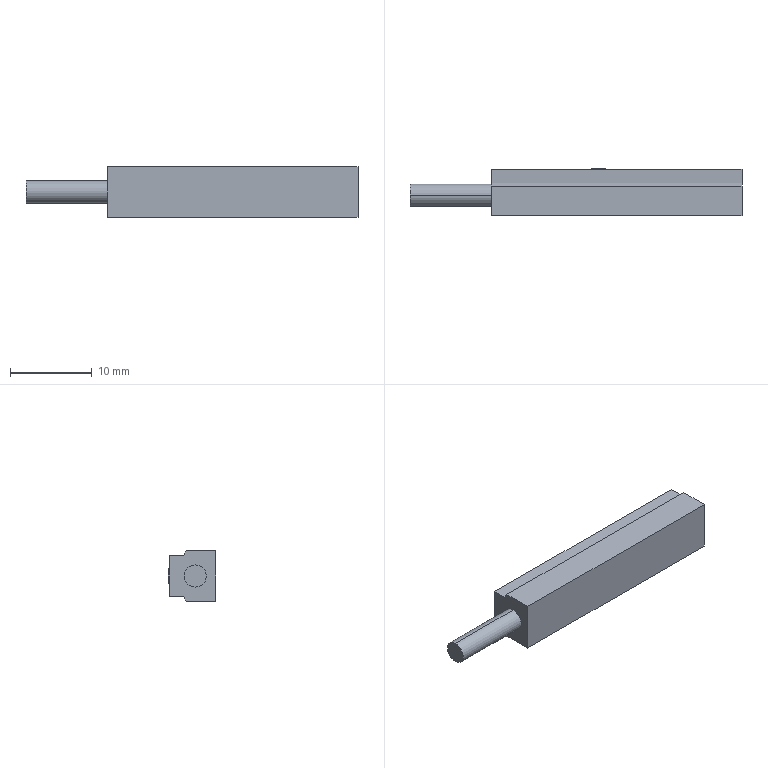Component | SolidWorks | F-YBExport-1-1_F-YBXCXSM10-15-Z73L-1_F-YBXCXSM10-15-Z73L_CXSSwitches(Z73)-1 | 1 solid | 33 faces | box 40.5 x 5.8 x 6.2 mm | volume 1063 mm3 | plane 27 | cylinder 6 | commonest cylinder face diameters 2.347 x2 2.5 x2 2.7 x2
STEP:
#1=COLOUR_RGB('',0.7922,0.8196,0.9333);
#2=FILL_AREA_STYLE_COLOUR('',#1);
#3=FILL_AREA_STYLE('',(#2));
#4=SURFACE_STYLE_FILL_AREA(#3);
#5=SURFACE_SIDE_STYLE('',(#4));
#6=SURFACE_STYLE_USAGE(.BOTH.,#5);
#7=PRESENTATION_STYLE_ASSIGNMENT((#6));
#8=CARTESIAN_POINT('',(13.609,14.688,6.265));
#9=VERTEX_POINT('',#8);
#10=CARTESIAN_POINT('',(13.537,14.688,6.227));
#11=VERTEX_POINT('',#10);
#12=CARTESIAN_POINT('',(13.563,14.688,6.265));
#13=DIRECTION('',(-0.,1.,0.));
#14=DIRECTION('',(1.,0.,0.));
#15=AXIS2_PLACEMENT_3D('',#12,#13,#14);
#16=CIRCLE('',#15,0.04621);
#17=EDGE_CURVE('',#9,#11,#16,.T.);
#18=ORIENTED_EDGE('',*,*,#17,.F.);
#19=CARTESIAN_POINT('',(13.609,14.648,6.265));
#20=VERTEX_POINT('',#19);
#21=CARTESIAN_POINT('',(13.609,14.688,6.265));
#22=DIRECTION('',(0.,-1.,-0.));
#23=VECTOR('',#22,39.37);
#24=LINE('',#21,#23);
#25=EDGE_CURVE('',#9,#20,#24,.T.);
#26=ORIENTED_EDGE('',*,*,#25,.T.);
#27=CARTESIAN_POINT('',(13.517,14.648,6.265));
#28=VERTEX_POINT('',#27);
#29=CARTESIAN_POINT('',(13.563,14.648,6.265));
#30=DIRECTION('',(-0.,1.,0.));
#31=DIRECTION('',(1.,0.,0.));
#32=AXIS2_PLACEMENT_3D('',#29,#30,#31);
#33=CIRCLE('',#32,0.04621);
#34=EDGE_CURVE('',#20,#28,#33,.T.);
#35=ORIENTED_EDGE('',*,*,#34,.T.);
#36=CARTESIAN_POINT('',(13.517,14.688,6.265));
#37=VERTEX_POINT('',#36);
#38=CARTESIAN_POINT('',(13.517,14.688,6.265));
#39=DIRECTION('',(0.,-1.,-0.));
#40=VECTOR('',#39,39.37);
#41=LINE('',#38,#40);
#42=EDGE_CURVE('',#37,#28,#41,.T.);
#43=ORIENTED_EDGE('',*,*,#42,.F.);
#44=CARTESIAN_POINT('',(13.525,14.688,6.239));
#45=VERTEX_POINT('',#44);
#46=CARTESIAN_POINT('',(13.563,14.688,6.265));
#47=DIRECTION('',(-0.,1.,0.));
#48=DIRECTION('',(1.,0.,0.));
#49=AXIS2_PLACEMENT_3D('',#46,#47,#48);
#50=CIRCLE('',#49,0.04621);
#51=EDGE_CURVE('',#45,#37,#50,.T.);
#52=ORIENTED_EDGE('',*,*,#51,.F.);
#53=CARTESIAN_POINT('',(13.525,14.668,6.239));
#54=VERTEX_POINT('',#53);
#55=CARTESIAN_POINT('',(13.525,14.688,6.239));
#56=DIRECTION('',(0.,-1.,-0.));
#57=VECTOR('',#56,39.37);
#58=LINE('',#55,#57);
#59=EDGE_CURVE('',#45,#54,#58,.T.);
#60=ORIENTED_EDGE('',*,*,#59,.T.);
#61=CARTESIAN_POINT('',(13.537,14.668,6.227));
#62=VERTEX_POINT('',#61);
#63=CARTESIAN_POINT('',(13.563,14.668,6.265));
#64=DIRECTION('',(-0.,1.,0.));
#65=DIRECTION('',(1.,0.,0.));
#66=AXIS2_PLACEMENT_3D('',#63,#64,#65);
#67=CIRCLE('',#66,0.04621);
#68=EDGE_CURVE('',#62,#54,#67,.T.);
#69=ORIENTED_EDGE('',*,*,#68,.F.);
#70=CARTESIAN_POINT('',(13.537,14.688,6.227));
#71=DIRECTION('',(-0.,1.,0.));
#72=VECTOR('',#71,39.37);
#73=LINE('',#70,#72);
#74=EDGE_CURVE('',#62,#11,#73,.T.);
#75=ORIENTED_EDGE('',*,*,#74,.T.);
#76=EDGE_LOOP('',(#18,#26,#35,#43,#52,#60,#69,#75));
#77=FACE_OUTER_BOUND('',#76,.T.);
#78=CARTESIAN_POINT('',(13.563,14.688,6.265));
#79=DIRECTION('',(0.,-1.,-0.));
#80=DIRECTION('',(-1.,0.,0.));
#81=AXIS2_PLACEMENT_3D('',#78,#79,#80);
#82=CYLINDRICAL_SURFACE('',#81,0.04621);
#83=ADVANCED_FACE('',(#77),#82,.T.);
#84=CARTESIAN_POINT('',(13.514,14.648,6.265));
#85=VERTEX_POINT('',#84);
#86=CARTESIAN_POINT('',(13.612,14.648,6.265));
#87=VERTEX_POINT('',#86);
#88=CARTESIAN_POINT('',(13.563,14.648,6.265));
#89=DIRECTION('',(-0.,1.,0.));
#90=DIRECTION('',(1.,0.,0.));
#91=AXIS2_PLACEMENT_3D('',#88,#89,#90);
#92=CIRCLE('',#91,0.04921);
#93=EDGE_CURVE('',#85,#87,#92,.T.);
#94=ORIENTED_EDGE('',*,*,#93,.F.);
#95=CARTESIAN_POINT('',(13.514,14.688,6.265));
#96=VERTEX_POINT('',#95);
#97=CARTESIAN_POINT('',(13.514,14.648,6.265));
#98=DIRECTION('',(-0.,1.,0.));
#99=VECTOR('',#98,39.37);
#100=LINE('',#97,#99);
#101=EDGE_CURVE('',#85,#96,#100,.T.);
#102=ORIENTED_EDGE('',*,*,#101,.T.);
#103=CARTESIAN_POINT('',(13.612,14.688,6.265));
#104=VERTEX_POINT('',#103);
#105=CARTESIAN_POINT('',(13.563,14.688,6.265));
#106=DIRECTION('',(-0.,1.,0.));
#107=DIRECTION('',(1.,0.,0.));
#108=AXIS2_PLACEMENT_3D('',#105,#106,#107);
#109=CIRCLE('',#108,0.04921);
#110=EDGE_CURVE('',#96,#104,#109,.T.);
#111=ORIENTED_EDGE('',*,*,#110,.T.);
#112=CARTESIAN_POINT('',(13.612,14.648,6.265));
#113=DIRECTION('',(-0.,1.,0.));
#114=VECTOR('',#113,39.37);
#115=LINE('',#112,#114);
#116=EDGE_CURVE('',#87,#104,#115,.T.);
#117=ORIENTED_EDGE('',*,*,#116,.F.);
#118=EDGE_LOOP('',(#94,#102,#111,#117));
#119=FACE_OUTER_BOUND('',#118,.T.);
#120=CARTESIAN_POINT('',(13.563,14.648,6.265));
#121=DIRECTION('',(-0.,1.,0.));
#122=DIRECTION('',(1.,0.,0.));
#123=AXIS2_PLACEMENT_3D('',#120,#121,#122);
#124=CYLINDRICAL_SURFACE('',#123,0.04921);
#125=ADVANCED_FACE('',(#119),#124,.F.);
#126=CARTESIAN_POINT('',(12.059,14.562,6.318));
#127=VERTEX_POINT('',#126);
#128=CARTESIAN_POINT('',(12.059,14.562,6.212));
#129=VERTEX_POINT('',#128);
#130=CARTESIAN_POINT('',(12.059,14.562,6.265));
#131=DIRECTION('',(-1.,-0.,-0.));
#132=DIRECTION('',(0.,0.,1.));
#133=AXIS2_PLACEMENT_3D('',#130,#131,#132);
#134=CIRCLE('',#133,0.05315);
#135=EDGE_CURVE('',#127,#129,#134,.T.);
#136=ORIENTED_EDGE('',*,*,#135,.F.);
#137=CARTESIAN_POINT('',(12.453,14.562,6.318));
#138=VERTEX_POINT('',#137);
#139=CARTESIAN_POINT('',(12.059,14.562,6.318));
#140=DIRECTION('',(1.,0.,0.));
#141=VECTOR('',#140,39.37);
#142=LINE('',#139,#141);
#143=EDGE_CURVE('',#127,#138,#142,.T.);
#144=ORIENTED_EDGE('',*,*,#143,.T.);
#145=CARTESIAN_POINT('',(12.453,14.562,6.212));
#146=VERTEX_POINT('',#145);
#147=CARTESIAN_POINT('',(12.453,14.562,6.265));
#148=DIRECTION('',(-1.,-0.,-0.));
#149=DIRECTION('',(0.,0.,-1.));
#150=AXIS2_PLACEMENT_3D('',#147,#148,#149);
#151=CIRCLE('',#150,0.05315);
#152=EDGE_CURVE('',#138,#146,#151,.T.);
#153=ORIENTED_EDGE('',*,*,#152,.T.);
#154=CARTESIAN_POINT('',(12.059,14.562,6.212));
#155=DIRECTION('',(1.,0.,0.));
#156=VECTOR('',#155,39.37);
#157=LINE('',#154,#156);
#158=EDGE_CURVE('',#129,#146,#157,.T.);
#159=ORIENTED_EDGE('',*,*,#158,.F.);
#160=EDGE_LOOP('',(#136,#144,#153,#159));
#161=FACE_OUTER_BOUND('',#160,.T.);
#162=CARTESIAN_POINT('',(12.059,14.562,6.265));
#163=DIRECTION('',(1.,0.,0.));
#164=DIRECTION('',(0.,0.,-1.));
#165=AXIS2_PLACEMENT_3D('',#162,#163,#164);
#166=CYLINDRICAL_SURFACE('',#165,0.05315);
#167=ADVANCED_FACE('',(#161),#166,.T.);
#168=CARTESIAN_POINT('',(12.925,14.668,6.304));
#169=VERTEX_POINT('',#168);
#170=CARTESIAN_POINT('',(13.004,14.668,6.304));
#171=VERTEX_POINT('',#170);
#172=CARTESIAN_POINT('',(13.004,14.668,6.304));
#173=DIRECTION('',(1.,0.,0.));
#174=VECTOR('',#173,39.37);
#175=LINE('',#172,#174);
#176=EDGE_CURVE('',#169,#171,#175,.T.);
#177=ORIENTED_EDGE('',*,*,#176,.T.);
#178=CARTESIAN_POINT('',(13.004,14.668,6.226));
#179=VERTEX_POINT('',#178);
#180=CARTESIAN_POINT('',(13.004,14.668,6.304));
#181=DIRECTION('',(0.,0.,-1.));
#182=VECTOR('',#181,39.37);
#183=LINE('',#180,#182);
#184=EDGE_CURVE('',#171,#179,#183,.T.);
#185=ORIENTED_EDGE('',*,*,#184,.T.);
#186=CARTESIAN_POINT('',(12.925,14.668,6.226));
#187=VERTEX_POINT('',#186);
#188=CARTESIAN_POINT('',(13.004,14.668,6.226));
#189=DIRECTION('',(-1.,-0.,-0.));
#190=VECTOR('',#189,39.37);
#191=LINE('',#188,#190);
#192=EDGE_CURVE('',#179,#187,#191,.T.);
#193=ORIENTED_EDGE('',*,*,#192,.T.);
#194=CARTESIAN_POINT('',(12.925,14.668,6.304));
#195=DIRECTION('',(-0.,-0.,1.));
#196=VECTOR('',#195,39.37);
#197=LINE('',#194,#196);
#198=EDGE_CURVE('',#187,#169,#197,.T.);
#199=ORIENTED_EDGE('',*,*,#198,.T.);
#200=EDGE_LOOP('',(#177,#185,#193,#199));
#201=FACE_OUTER_BOUND('',#200,.T.);
#202=CARTESIAN_POINT('',(12.93,14.668,6.299));
#203=VERTEX_POINT('',#202);
#204=CARTESIAN_POINT('',(12.999,14.668,6.299));
#205=VERTEX_POINT('',#204);
#206=CARTESIAN_POINT('',(12.93,14.668,6.299));
#207=DIRECTION('',(1.,0.,0.));
#208=VECTOR('',#207,39.37);
#209=LINE('',#206,#208);
#210=EDGE_CURVE('',#203,#205,#209,.T.);
#211=ORIENTED_EDGE('',*,*,#210,.F.);
#212=CARTESIAN_POINT('',(12.93,14.668,6.23));
#213=VERTEX_POINT('',#212);
#214=CARTESIAN_POINT('',(12.93,14.668,6.299));
#215=DIRECTION('',(-0.,-0.,1.));
#216=VECTOR('',#215,39.37);
#217=LINE('',#214,#216);
#218=EDGE_CURVE('',#213,#203,#217,.T.);
#219=ORIENTED_EDGE('',*,*,#218,.F.);
#220=CARTESIAN_POINT('',(12.999,14.668,6.23));
#221=VERTEX_POINT('',#220);
#222=CARTESIAN_POINT('',(12.93,14.668,6.23));
#223=DIRECTION('',(-1.,-0.,-0.));
#224=VECTOR('',#223,39.37);
#225=LINE('',#222,#224);
#226=EDGE_CURVE('',#221,#213,#225,.T.);
#227=ORIENTED_EDGE('',*,*,#226,.F.);
#228=CARTESIAN_POINT('',(12.999,14.668,6.299));
#229=DIRECTION('',(0.,0.,-1.));
#230=VECTOR('',#229,39.37);
#231=LINE('',#228,#230);
#232=EDGE_CURVE('',#205,#221,#231,.T.);
#233=ORIENTED_EDGE('',*,*,#232,.F.);
#234=EDGE_LOOP('',(#211,#219,#227,#233));
#235=FACE_BOUND('',#234,.T.);
#236=CARTESIAN_POINT('',(12.925,14.668,6.304));
#237=DIRECTION('',(0.,-1.,-0.));
#238=DIRECTION('',(-1.,-0.,-0.));
#239=AXIS2_PLACEMENT_3D('',#236,#237,#238);
#240=PLANE('',#239);
#241=ADVANCED_FACE('',(#201,#235),#240,.F.);
#242=CARTESIAN_POINT('',(13.602,14.688,6.291));
#243=VERTEX_POINT('',#242);
#244=CARTESIAN_POINT('',(13.569,14.688,6.259));
#245=DIRECTION('',(-0.7071,0.,-0.7071));
#246=VECTOR('',#245,39.37);
#247=LINE('',#244,#246);
#248=EDGE_CURVE('',#243,#11,#247,.T.);
#249=ORIENTED_EDGE('',*,*,#248,.F.);
#250=CARTESIAN_POINT('',(13.563,14.688,6.265));
#251=DIRECTION('',(-0.,1.,0.));
#252=DIRECTION('',(1.,0.,0.));
#253=AXIS2_PLACEMENT_3D('',#250,#251,#252);
#254=CIRCLE('',#253,0.04621);
#255=EDGE_CURVE('',#243,#9,#254,.T.);
#256=ORIENTED_EDGE('',*,*,#255,.T.);
#257=ORIENTED_EDGE('',*,*,#17,.T.);
#258=EDGE_LOOP('',(#249,#256,#257));
#259=FACE_OUTER_BOUND('',#258,.T.);
#260=CARTESIAN_POINT('',(13.563,14.688,6.265));
#261=DIRECTION('',(-0.,1.,0.));
#262=DIRECTION('',(1.,0.,0.));
#263=AXIS2_PLACEMENT_3D('',#260,#261,#262);
#264=PLANE('',#263);
#265=ADVANCED_FACE('',(#259),#264,.T.);
#266=CARTESIAN_POINT('',(13.563,14.648,6.265));
#267=DIRECTION('',(-0.,1.,0.));
#268=DIRECTION('',(1.,0.,0.));
#269=AXIS2_PLACEMENT_3D('',#266,#267,#268);
#270=CIRCLE('',#269,0.04921);
#271=EDGE_CURVE('',#87,#85,#270,.T.);
#272=ORIENTED_EDGE('',*,*,#271,.T.);
#273=ORIENTED_EDGE('',*,*,#93,.T.);
#274=EDGE_LOOP('',(#272,#273));
#275=FACE_OUTER_BOUND('',#274,.T.);
#276=CARTESIAN_POINT('',(13.563,14.648,6.265));
#277=DIRECTION('',(-0.,1.,0.));
#278=DIRECTION('',(1.,0.,0.));
#279=AXIS2_PLACEMENT_3D('',#276,#277,#278);
#280=CIRCLE('',#279,0.04621);
#281=EDGE_CURVE('',#28,#20,#280,.T.);
#282=ORIENTED_EDGE('',*,*,#281,.F.);
#283=ORIENTED_EDGE('',*,*,#34,.F.);
#284=EDGE_LOOP('',(#282,#283));
#285=FACE_BOUND('',#284,.T.);
#286=CARTESIAN_POINT('',(13.563,14.648,6.265));
#287=DIRECTION('',(-0.,1.,0.));
#288=DIRECTION('',(1.,0.,0.));
#289=AXIS2_PLACEMENT_3D('',#286,#287,#288);
#290=PLANE('',#289);
#291=ADVANCED_FACE('',(#275,#285),#290,.T.);
#292=CARTESIAN_POINT('',(12.453,14.464,6.143));
#293=VERTEX_POINT('',#292);
#294=CARTESIAN_POINT('',(12.453,14.605,6.143));
#295=VERTEX_POINT('',#294);
#296=CARTESIAN_POINT('',(12.453,14.464,6.143));
#297=DIRECTION('',(-0.,1.,0.));
#298=VECTOR('',#297,39.37);
#299=LINE('',#296,#298);
#300=EDGE_CURVE('',#293,#295,#299,.T.);
#301=ORIENTED_EDGE('',*,*,#300,.F.);
#302=CARTESIAN_POINT('',(12.453,14.464,6.387));
#303=VERTEX_POINT('',#302);
#304=CARTESIAN_POINT('',(12.453,14.464,6.387));
#305=DIRECTION('',(0.,0.,-1.));
#306=VECTOR('',#305,39.37);
#307=LINE('',#304,#306);
#308=EDGE_CURVE('',#303,#293,#307,.T.);
#309=ORIENTED_EDGE('',*,*,#308,.F.);
#310=CARTESIAN_POINT('',(12.453,14.605,6.387));
#311=VERTEX_POINT('',#310);
#312=CARTESIAN_POINT('',(12.453,14.464,6.387));
#313=DIRECTION('',(0.,-1.,-0.));
#314=VECTOR('',#313,39.37);
#315=LINE('',#312,#314);
#316=EDGE_CURVE('',#311,#303,#315,.T.);
#317=ORIENTED_EDGE('',*,*,#316,.F.);
#318=CARTESIAN_POINT('',(12.453,14.619,6.363));
#319=VERTEX_POINT('',#318);
#320=CARTESIAN_POINT('',(12.453,14.605,6.387));
#321=DIRECTION('',(-0.,-0.5,0.866));
#322=VECTOR('',#321,39.37);
#323=LINE('',#320,#322);
#324=EDGE_CURVE('',#319,#311,#323,.T.);
#325=ORIENTED_EDGE('',*,*,#324,.F.);
#326=CARTESIAN_POINT('',(12.453,14.688,6.363));
#327=VERTEX_POINT('',#326);
#328=CARTESIAN_POINT('',(12.453,14.619,6.363));
#329=DIRECTION('',(0.,-1.,-0.));
#330=VECTOR('',#329,39.37);
#331=LINE('',#328,#330);
#332=EDGE_CURVE('',#327,#319,#331,.T.);
#333=ORIENTED_EDGE('',*,*,#332,.F.);
#334=CARTESIAN_POINT('',(12.453,14.688,6.167));
#335=VERTEX_POINT('',#334);
#336=CARTESIAN_POINT('',(12.453,14.688,6.167));
#337=DIRECTION('',(-0.,-0.,1.));
#338=VECTOR('',#337,39.37);
#339=LINE('',#336,#338);
#340=EDGE_CURVE('',#335,#327,#339,.T.);
#341=ORIENTED_EDGE('',*,*,#340,.F.);
#342=CARTESIAN_POINT('',(12.453,14.619,6.167));
#343=VERTEX_POINT('',#342);
#344=CARTESIAN_POINT('',(12.453,14.619,6.167));
#345=DIRECTION('',(0.,1.,-0.));
#346=VECTOR('',#345,39.37);
#347=LINE('',#344,#346);
#348=EDGE_CURVE('',#343,#335,#347,.T.);
#349=ORIENTED_EDGE('',*,*,#348,.F.);
#350=CARTESIAN_POINT('',(12.453,14.605,6.143));
#351=DIRECTION('',(-0.,0.5,0.866));
#352=VECTOR('',#351,39.37);
#353=LINE('',#350,#352);
#354=EDGE_CURVE('',#295,#343,#353,.T.);
#355=ORIENTED_EDGE('',*,*,#354,.F.);
#356=EDGE_LOOP('',(#301,#309,#317,#325,#333,#341,#349,#355));
#357=FACE_OUTER_BOUND('',#356,.T.);
#358=CARTESIAN_POINT('',(12.453,14.562,6.265));
#359=DIRECTION('',(-1.,-0.,-0.));
#360=DIRECTION('',(0.,0.,-1.));
#361=AXIS2_PLACEMENT_3D('',#358,#359,#360);
#362=CIRCLE('',#361,0.05315);
#363=EDGE_CURVE('',#146,#138,#362,.T.);
#364=ORIENTED_EDGE('',*,*,#363,.F.);
#365=ORIENTED_EDGE('',*,*,#152,.F.);
#366=EDGE_LOOP('',(#364,#365));
#367=FACE_BOUND('',#366,.T.);
#368=CARTESIAN_POINT('',(12.453,14.688,6.143));
#369=DIRECTION('',(1.,0.,0.));
#370=DIRECTION('',(0.,0.,-1.));
#371=AXIS2_PLACEMENT_3D('',#368,#369,#370);
#372=PLANE('',#371);
#373=ADVANCED_FACE('',(#357,#367),#372,.F.);
#374=CARTESIAN_POINT('',(13.654,14.464,6.143));
#375=VERTEX_POINT('',#374);
#376=CARTESIAN_POINT('',(13.654,14.605,6.143));
#377=VERTEX_POINT('',#376);
#378=CARTESIAN_POINT('',(13.654,14.464,6.143));
#379=DIRECTION('',(-0.,1.,0.));
#380=VECTOR('',#379,39.37);
#381=LINE('',#378,#380);
#382=EDGE_CURVE('',#375,#377,#381,.T.);
#383=ORIENTED_EDGE('',*,*,#382,.F.);
#384=CARTESIAN_POINT('',(12.453,14.464,6.143));
#385=DIRECTION('',(1.,0.,0.));
#386=VECTOR('',#385,39.37);
#387=LINE('',#384,#386);
#388=EDGE_CURVE('',#293,#375,#387,.T.);
#389=ORIENTED_EDGE('',*,*,#388,.F.);
#390=ORIENTED_EDGE('',*,*,#300,.T.);
#391=CARTESIAN_POINT('',(12.453,14.605,6.143));
#392=DIRECTION('',(1.,0.,0.));
#393=VECTOR('',#392,39.37);
#394=LINE('',#391,#393);
#395=EDGE_CURVE('',#295,#377,#394,.T.);
#396=ORIENTED_EDGE('',*,*,#395,.T.);
#397=EDGE_LOOP('',(#383,#389,#390,#396));
#398=FACE_OUTER_BOUND('',#397,.T.);
#399=CARTESIAN_POINT('',(12.453,14.464,6.143));
#400=DIRECTION('',(0.,0.,-1.));
#401=DIRECTION('',(-1.,-0.,-0.));
#402=AXIS2_PLACEMENT_3D('',#399,#400,#401);
#403=PLANE('',#402);
#404=ADVANCED_FACE('',(#398),#403,.T.);
#405=CARTESIAN_POINT('',(13.654,14.464,6.387));
#406=VERTEX_POINT('',#405);
#407=CARTESIAN_POINT('',(13.654,14.464,6.387));
#408=DIRECTION('',(0.,0.,-1.));
#409=VECTOR('',#408,39.37);
#410=LINE('',#407,#409);
#411=EDGE_CURVE('',#406,#375,#410,.T.);
#412=ORIENTED_EDGE('',*,*,#411,.F.);
#413=CARTESIAN_POINT('',(12.453,14.464,6.387));
#414=DIRECTION('',(1.,0.,0.));
#415=VECTOR('',#414,39.37);
#416=LINE('',#413,#415);
#417=EDGE_CURVE('',#303,#406,#416,.T.);
#418=ORIENTED_EDGE('',*,*,#417,.F.);
#419=ORIENTED_EDGE('',*,*,#308,.T.);
#420=ORIENTED_EDGE('',*,*,#388,.T.);
#421=EDGE_LOOP('',(#412,#418,#419,#420));
#422=FACE_OUTER_BOUND('',#421,.T.);
#423=CARTESIAN_POINT('',(12.453,14.464,6.387));
#424=DIRECTION('',(0.,-1.,-0.));
#425=DIRECTION('',(-1.,-0.,-0.));
#426=AXIS2_PLACEMENT_3D('',#423,#424,#425);
#427=PLANE('',#426);
#428=ADVANCED_FACE('',(#422),#427,.T.);
#429=CARTESIAN_POINT('',(13.654,14.605,6.387));
#430=VERTEX_POINT('',#429);
#431=CARTESIAN_POINT('',(13.654,14.464,6.387));
#432=DIRECTION('',(0.,-1.,-0.));
#433=VECTOR('',#432,39.37);
#434=LINE('',#431,#433);
#435=EDGE_CURVE('',#430,#406,#434,.T.);
#436=ORIENTED_EDGE('',*,*,#435,.F.);
#437=CARTESIAN_POINT('',(12.453,14.605,6.387));
#438=DIRECTION('',(1.,0.,0.));
#439=VECTOR('',#438,39.37);
#440=LINE('',#437,#439);
#441=EDGE_CURVE('',#311,#430,#440,.T.);
#442=ORIENTED_EDGE('',*,*,#441,.F.);
#443=ORIENTED_EDGE('',*,*,#316,.T.);
#444=ORIENTED_EDGE('',*,*,#417,.T.);
#445=EDGE_LOOP('',(#436,#442,#443,#444));
#446=FACE_OUTER_BOUND('',#445,.T.);
#447=CARTESIAN_POINT('',(12.453,14.464,6.387));
#448=DIRECTION('',(-0.,-0.,1.));
#449=DIRECTION('',(1.,0.,0.));
#450=AXIS2_PLACEMENT_3D('',#447,#448,#449);
#451=PLANE('',#450);
#452=ADVANCED_FACE('',(#446),#451,.T.);
#453=CARTESIAN_POINT('',(13.654,14.619,6.363));
#454=VERTEX_POINT('',#453);
#455=CARTESIAN_POINT('',(13.654,14.605,6.387));
#456=DIRECTION('',(-0.,-0.5,0.866));
#457=VECTOR('',#456,39.37);
#458=LINE('',#455,#457);
#459=EDGE_CURVE('',#454,#430,#458,.T.);
#460=ORIENTED_EDGE('',*,*,#459,.F.);
#461=CARTESIAN_POINT('',(12.453,14.619,6.363));
#462=DIRECTION('',(1.,0.,0.));
#463=VECTOR('',#462,39.37);
#464=LINE('',#461,#463);
#465=EDGE_CURVE('',#319,#454,#464,.T.);
#466=ORIENTED_EDGE('',*,*,#465,.F.);
#467=ORIENTED_EDGE('',*,*,#324,.T.);
#468=ORIENTED_EDGE('',*,*,#441,.T.);
#469=EDGE_LOOP('',(#460,#466,#467,#468));
#470=FACE_OUTER_BOUND('',#469,.T.);
#471=CARTESIAN_POINT('',(12.453,14.605,6.387));
#472=DIRECTION('',(-0.,0.866,0.5));
#473=DIRECTION('',(-0.,-0.5,0.866));
#474=AXIS2_PLACEMENT_3D('',#471,#472,#473);
#475=PLANE('',#474);
#476=ADVANCED_FACE('',(#470),#475,.T.);
#477=CARTESIAN_POINT('',(13.654,14.688,6.363));
#478=VERTEX_POINT('',#477);
#479=CARTESIAN_POINT('',(13.654,14.619,6.363));
#480=DIRECTION('',(0.,-1.,-0.));
#481=VECTOR('',#480,39.37);
#482=LINE('',#479,#481);
#483=EDGE_CURVE('',#478,#454,#482,.T.);
#484=ORIENTED_EDGE('',*,*,#483,.F.);
#485=CARTESIAN_POINT('',(12.453,14.688,6.363));
#486=DIRECTION('',(1.,0.,0.));
#487=VECTOR('',#486,39.37);
#488=LINE('',#485,#487);
#489=EDGE_CURVE('',#327,#478,#488,.T.);
#490=ORIENTED_EDGE('',*,*,#489,.F.);
#491=ORIENTED_EDGE('',*,*,#332,.T.);
#492=ORIENTED_EDGE('',*,*,#465,.T.);
#493=EDGE_LOOP('',(#484,#490,#491,#492));
#494=FACE_OUTER_BOUND('',#493,.T.);
#495=CARTESIAN_POINT('',(12.453,14.619,6.363));
#496=DIRECTION('',(-0.,-0.,1.));
#497=DIRECTION('',(1.,0.,0.));
#498=AXIS2_PLACEMENT_3D('',#495,#496,#497);
#499=PLANE('',#498);
#500=ADVANCED_FACE('',(#494),#499,.T.);
#501=CARTESIAN_POINT('',(12.925,14.688,6.304));
#502=VERTEX_POINT('',#501);
#503=CARTESIAN_POINT('',(13.004,14.688,6.304));
#504=VERTEX_POINT('',#503);
#505=CARTESIAN_POINT('',(13.004,14.688,6.304));
#506=DIRECTION('',(1.,0.,0.));
#507=VECTOR('',#506,39.37);
#508=LINE('',#505,#507);
#509=EDGE_CURVE('',#502,#504,#508,.T.);
#510=ORIENTED_EDGE('',*,*,#509,.F.);
#511=CARTESIAN_POINT('',(12.925,14.688,6.226));
#512=VERTEX_POINT('',#511);
#513=CARTESIAN_POINT('',(12.925,14.688,6.304));
#514=DIRECTION('',(-0.,-0.,1.));
#515=VECTOR('',#514,39.37);
#516=LINE('',#513,#515);
#517=EDGE_CURVE('',#512,#502,#516,.T.);
#518=ORIENTED_EDGE('',*,*,#517,.F.);
#519=CARTESIAN_POINT('',(13.004,14.688,6.226));
#520=VERTEX_POINT('',#519);
#521=CARTESIAN_POINT('',(13.004,14.688,6.226));
#522=DIRECTION('',(-1.,-0.,-0.));
#523=VECTOR('',#522,39.37);
#524=LINE('',#521,#523);
#525=EDGE_CURVE('',#520,#512,#524,.T.);
#526=ORIENTED_EDGE('',*,*,#525,.F.);
#527=CARTESIAN_POINT('',(13.004,14.688,6.304));
#528=DIRECTION('',(0.,0.,-1.));
#529=VECTOR('',#528,39.37);
#530=LINE('',#527,#529);
#531=EDGE_CURVE('',#504,#520,#530,.T.);
#532=ORIENTED_EDGE('',*,*,#531,.F.);
#533=EDGE_LOOP('',(#510,#518,#526,#532));
#534=FACE_BOUND('',#533,.T.);
#535=CARTESIAN_POINT('',(13.563,14.688,6.265));
#536=DIRECTION('',(-0.,1.,0.));
#537=DIRECTION('',(1.,0.,0.));
#538=AXIS2_PLACEMENT_3D('',#535,#536,#537);
#539=CIRCLE('',#538,0.04921);
#540=EDGE_CURVE('',#104,#96,#539,.T.);
#541=ORIENTED_EDGE('',*,*,#540,.F.);
#542=ORIENTED_EDGE('',*,*,#110,.F.);
#543=EDGE_LOOP('',(#541,#542));
#544=FACE_BOUND('',#543,.T.);
#545=CARTESIAN_POINT('',(13.654,14.688,6.167));
#546=VERTEX_POINT('',#545);
#547=CARTESIAN_POINT('',(13.654,14.688,6.167));
#548=DIRECTION('',(-0.,-0.,1.));
#549=VECTOR('',#548,39.37);
#550=LINE('',#547,#549);
#551=EDGE_CURVE('',#546,#478,#550,.T.);
#552=ORIENTED_EDGE('',*,*,#551,.F.);
#553=CARTESIAN_POINT('',(12.453,14.688,6.167));
#554=DIRECTION('',(1.,0.,0.));
#555=VECTOR('',#554,39.37);
#556=LINE('',#553,#555);
#557=EDGE_CURVE('',#335,#546,#556,.T.);
#558=ORIENTED_EDGE('',*,*,#557,.F.);
#559=ORIENTED_EDGE('',*,*,#340,.T.);
#560=ORIENTED_EDGE('',*,*,#489,.T.);
#561=EDGE_LOOP('',(#552,#558,#559,#560));
#562=FACE_OUTER_BOUND('',#561,.T.);
#563=CARTESIAN_POINT('',(12.453,14.688,6.167));
#564=DIRECTION('',(-0.,1.,0.));
#565=DIRECTION('',(1.,0.,0.));
#566=AXIS2_PLACEMENT_3D('',#563,#564,#565);
#567=PLANE('',#566);
#568=ADVANCED_FACE('',(#534,#544,#562),#567,.T.);
#569=CARTESIAN_POINT('',(13.654,14.619,6.167));
#570=VERTEX_POINT('',#569);
#571=CARTESIAN_POINT('',(13.654,14.619,6.167));
#572=DIRECTION('',(0.,1.,-0.));
#573=VECTOR('',#572,39.37);
#574=LINE('',#571,#573);
#575=EDGE_CURVE('',#570,#546,#574,.T.);
#576=ORIENTED_EDGE('',*,*,#575,.F.);
#577=CARTESIAN_POINT('',(12.453,14.619,6.167));
#578=DIRECTION('',(1.,0.,0.));
#579=VECTOR('',#578,39.37);
#580=LINE('',#577,#579);
#581=EDGE_CURVE('',#343,#570,#580,.T.);
#582=ORIENTED_EDGE('',*,*,#581,.F.);
#583=ORIENTED_EDGE('',*,*,#348,.T.);
#584=ORIENTED_EDGE('',*,*,#557,.T.);
#585=EDGE_LOOP('',(#576,#582,#583,#584));
#586=FACE_OUTER_BOUND('',#585,.T.);
#587=CARTESIAN_POINT('',(12.453,14.619,6.167));
#588=DIRECTION('',(0.,-0.,-1.));
#589=DIRECTION('',(0.,1.,-0.));
#590=AXIS2_PLACEMENT_3D('',#587,#588,#589);
#591=PLANE('',#590);
#592=ADVANCED_FACE('',(#586),#591,.T.);
#593=CARTESIAN_POINT('',(13.654,14.605,6.143));
#594=DIRECTION('',(-0.,0.5,0.866));
#595=VECTOR('',#594,39.37);
#596=LINE('',#593,#595);
#597=EDGE_CURVE('',#377,#570,#596,.T.);
#598=ORIENTED_EDGE('',*,*,#597,.F.);
#599=ORIENTED_EDGE('',*,*,#395,.F.);
#600=ORIENTED_EDGE('',*,*,#354,.T.);
#601=ORIENTED_EDGE('',*,*,#581,.T.);
#602=EDGE_LOOP('',(#598,#599,#600,#601));
#603=FACE_OUTER_BOUND('',#602,.T.);
#604=CARTESIAN_POINT('',(12.453,14.605,6.143));
#605=DIRECTION('',(0.,0.866,-0.5));
#606=DIRECTION('',(-0.,0.5,0.866));
#607=AXIS2_PLACEMENT_3D('',#604,#605,#606);
#608=PLANE('',#607);
#609=ADVANCED_FACE('',(#603),#608,.T.);
#610=ORIENTED_EDGE('',*,*,#382,.T.);
#611=ORIENTED_EDGE('',*,*,#597,.T.);
#612=ORIENTED_EDGE('',*,*,#575,.T.);
#613=ORIENTED_EDGE('',*,*,#551,.T.);
#614=ORIENTED_EDGE('',*,*,#483,.T.);
#615=ORIENTED_EDGE('',*,*,#459,.T.);
#616=ORIENTED_EDGE('',*,*,#435,.T.);
#617=ORIENTED_EDGE('',*,*,#411,.T.);
#618=EDGE_LOOP('',(#610,#611,#612,#613,#614,#615,#616,#617));
#619=FACE_OUTER_BOUND('',#618,.T.);
#620=CARTESIAN_POINT('',(13.654,14.688,6.143));
#621=DIRECTION('',(1.,0.,0.));
#622=DIRECTION('',(0.,0.,-1.));
#623=AXIS2_PLACEMENT_3D('',#620,#621,#622);
#624=PLANE('',#623);
#625=ADVANCED_FACE('',(#619),#624,.T.);
#626=ORIENTED_EDGE('',*,*,#143,.F.);
#627=CARTESIAN_POINT('',(12.059,14.562,6.265));
#628=DIRECTION('',(-1.,-0.,-0.));
#629=DIRECTION('',(0.,0.,1.));
#630=AXIS2_PLACEMENT_3D('',#627,#628,#629);
#631=CIRCLE('',#630,0.05315);
#632=EDGE_CURVE('',#129,#127,#631,.T.);
#633=ORIENTED_EDGE('',*,*,#632,.F.);
#634=ORIENTED_EDGE('',*,*,#158,.T.);
#635=ORIENTED_EDGE('',*,*,#363,.T.);
#636=EDGE_LOOP('',(#626,#633,#634,#635));
#637=FACE_OUTER_BOUND('',#636,.T.);
#638=CARTESIAN_POINT('',(12.059,14.562,6.265));
#639=DIRECTION('',(1.,0.,0.));
#640=DIRECTION('',(0.,0.,-1.));
#641=AXIS2_PLACEMENT_3D('',#638,#639,#640);
#642=CYLINDRICAL_SURFACE('',#641,0.05315);
#643=ADVANCED_FACE('',(#637),#642,.T.);
#644=ORIENTED_EDGE('',*,*,#632,.T.);
#645=ORIENTED_EDGE('',*,*,#135,.T.);
#646=EDGE_LOOP('',(#644,#645));
#647=FACE_OUTER_BOUND('',#646,.T.);
#648=CARTESIAN_POINT('',(12.059,14.562,6.265));
#649=DIRECTION('',(-1.,-0.,-0.));
#650=DIRECTION('',(-0.,-0.,1.));
#651=AXIS2_PLACEMENT_3D('',#648,#649,#650);
#652=PLANE('',#651);
#653=ADVANCED_FACE('',(#647),#652,.T.);
#654=ORIENTED_EDGE('',*,*,#101,.F.);
#655=ORIENTED_EDGE('',*,*,#271,.F.);
#656=ORIENTED_EDGE('',*,*,#116,.T.);
#657=ORIENTED_EDGE('',*,*,#540,.T.);
#658=EDGE_LOOP('',(#654,#655,#656,#657));
#659=FACE_OUTER_BOUND('',#658,.T.);
#660=CARTESIAN_POINT('',(13.563,14.648,6.265));
#661=DIRECTION('',(-0.,1.,0.));
#662=DIRECTION('',(1.,0.,0.));
#663=AXIS2_PLACEMENT_3D('',#660,#661,#662);
#664=CYLINDRICAL_SURFACE('',#663,0.04921);
#665=ADVANCED_FACE('',(#659),#664,.F.);
#666=ORIENTED_EDGE('',*,*,#25,.F.);
#667=ORIENTED_EDGE('',*,*,#255,.F.);
#668=CARTESIAN_POINT('',(13.602,14.668,6.291));
#669=VERTEX_POINT('',#668);
#670=CARTESIAN_POINT('',(13.602,14.688,6.291));
#671=DIRECTION('',(0.,-1.,-0.));
#672=VECTOR('',#671,39.37);
#673=LINE('',#670,#672);
#674=EDGE_CURVE('',#243,#669,#673,.T.);
#675=ORIENTED_EDGE('',*,*,#674,.T.);
#676=CARTESIAN_POINT('',(13.589,14.668,6.303));
#677=VERTEX_POINT('',#676);
#678=CARTESIAN_POINT('',(13.563,14.668,6.265));
#679=DIRECTION('',(-0.,1.,0.));
#680=DIRECTION('',(1.,0.,0.));
#681=AXIS2_PLACEMENT_3D('',#678,#679,#680);
#682=CIRCLE('',#681,0.04621);
#683=EDGE_CURVE('',#677,#669,#682,.T.);
#684=ORIENTED_EDGE('',*,*,#683,.F.);
#685=CARTESIAN_POINT('',(13.589,14.688,6.303));
#686=VERTEX_POINT('',#685);
#687=CARTESIAN_POINT('',(13.589,14.688,6.303));
#688=DIRECTION('',(-0.,1.,0.));
#689=VECTOR('',#688,39.37);
#690=LINE('',#687,#689);
#691=EDGE_CURVE('',#677,#686,#690,.T.);
#692=ORIENTED_EDGE('',*,*,#691,.T.);
#693=CARTESIAN_POINT('',(13.563,14.688,6.265));
#694=DIRECTION('',(-0.,1.,0.));
#695=DIRECTION('',(1.,0.,0.));
#696=AXIS2_PLACEMENT_3D('',#693,#694,#695);
#697=CIRCLE('',#696,0.04621);
#698=EDGE_CURVE('',#37,#686,#697,.T.);
#699=ORIENTED_EDGE('',*,*,#698,.F.);
#700=ORIENTED_EDGE('',*,*,#42,.T.);
#701=ORIENTED_EDGE('',*,*,#281,.T.);
#702=EDGE_LOOP('',(#666,#667,#675,#684,#692,#699,#700,#701));
#703=FACE_OUTER_BOUND('',#702,.T.);
#704=CARTESIAN_POINT('',(13.563,14.688,6.265));
#705=DIRECTION('',(0.,-1.,-0.));
#706=DIRECTION('',(-1.,0.,0.));
#707=AXIS2_PLACEMENT_3D('',#704,#705,#706);
#708=CYLINDRICAL_SURFACE('',#707,0.04621);
#709=ADVANCED_FACE('',(#703),#708,.T.);
#710=CARTESIAN_POINT('',(13.557,14.688,6.271));
#711=DIRECTION('',(0.7071,-0.,0.7071));
#712=VECTOR('',#711,39.37);
#713=LINE('',#710,#712);
#714=EDGE_CURVE('',#45,#686,#713,.T.);
#715=ORIENTED_EDGE('',*,*,#714,.F.);
#716=ORIENTED_EDGE('',*,*,#51,.T.);
#717=ORIENTED_EDGE('',*,*,#698,.T.);
#718=EDGE_LOOP('',(#715,#716,#717));
#719=FACE_OUTER_BOUND('',#718,.T.);
#720=CARTESIAN_POINT('',(13.563,14.688,6.265));
#721=DIRECTION('',(-0.,1.,0.));
#722=DIRECTION('',(1.,0.,0.));
#723=AXIS2_PLACEMENT_3D('',#720,#721,#722);
#724=PLANE('',#723);
#725=ADVANCED_FACE('',(#719),#724,.T.);
#726=ORIENTED_EDGE('',*,*,#68,.T.);
#727=CARTESIAN_POINT('',(13.525,14.668,6.239));
#728=DIRECTION('',(0.7071,-0.,0.7071));
#729=VECTOR('',#728,39.37);
#730=LINE('',#727,#729);
#731=EDGE_CURVE('',#54,#677,#730,.T.);
#732=ORIENTED_EDGE('',*,*,#731,.T.);
#733=ORIENTED_EDGE('',*,*,#683,.T.);
#734=CARTESIAN_POINT('',(13.537,14.668,6.227));
#735=DIRECTION('',(-0.7071,0.,-0.7071));
#736=VECTOR('',#735,39.37);
#737=LINE('',#734,#736);
#738=EDGE_CURVE('',#669,#62,#737,.T.);
#739=ORIENTED_EDGE('',*,*,#738,.T.);
#740=EDGE_LOOP('',(#726,#732,#733,#739));
#741=FACE_OUTER_BOUND('',#740,.T.);
#742=CARTESIAN_POINT('',(13.563,14.668,6.265));
#743=DIRECTION('',(-0.,1.,0.));
#744=DIRECTION('',(1.,0.,0.));
#745=AXIS2_PLACEMENT_3D('',#742,#743,#744);
#746=PLANE('',#745);
#747=ADVANCED_FACE('',(#741),#746,.T.);
#748=ORIENTED_EDGE('',*,*,#248,.T.);
#749=ORIENTED_EDGE('',*,*,#74,.F.);
#750=ORIENTED_EDGE('',*,*,#738,.F.);
#751=ORIENTED_EDGE('',*,*,#674,.F.);
#752=EDGE_LOOP('',(#748,#749,#750,#751));
#753=FACE_OUTER_BOUND('',#752,.T.);
#754=CARTESIAN_POINT('',(13.537,14.668,6.227));
#755=DIRECTION('',(0.7071,0.,-0.7071));
#756=DIRECTION('',(-0.7071,0.,-0.7071));
#757=AXIS2_PLACEMENT_3D('',#754,#755,#756);
#758=PLANE('',#757);
#759=ADVANCED_FACE('',(#753),#758,.F.);
#760=ORIENTED_EDGE('',*,*,#714,.T.);
#761=ORIENTED_EDGE('',*,*,#691,.F.);
#762=ORIENTED_EDGE('',*,*,#731,.F.);
#763=ORIENTED_EDGE('',*,*,#59,.F.);
#764=EDGE_LOOP('',(#760,#761,#762,#763));
#765=FACE_OUTER_BOUND('',#764,.T.);
#766=CARTESIAN_POINT('',(13.525,14.668,6.239));
#767=DIRECTION('',(-0.7071,-0.,0.7071));
#768=DIRECTION('',(0.7071,-0.,0.7071));
#769=AXIS2_PLACEMENT_3D('',#766,#767,#768);
#770=PLANE('',#769);
#771=ADVANCED_FACE('',(#765),#770,.F.);
#772=ORIENTED_EDGE('',*,*,#509,.T.);
#773=CARTESIAN_POINT('',(13.004,14.668,6.304));
#774=DIRECTION('',(-0.,1.,0.));
#775=VECTOR('',#774,39.37);
#776=LINE('',#773,#775);
#777=EDGE_CURVE('',#171,#504,#776,.T.);
#778=ORIENTED_EDGE('',*,*,#777,.F.);
#779=ORIENTED_EDGE('',*,*,#176,.F.);
#780=CARTESIAN_POINT('',(12.925,14.668,6.304));
#781=DIRECTION('',(-0.,1.,0.));
#782=VECTOR('',#781,39.37);
#783=LINE('',#780,#782);
#784=EDGE_CURVE('',#169,#502,#783,.T.);
#785=ORIENTED_EDGE('',*,*,#784,.T.);
#786=EDGE_LOOP('',(#772,#778,#779,#785));
#787=FACE_OUTER_BOUND('',#786,.T.);
#788=CARTESIAN_POINT('',(13.004,14.668,6.304));
#789=DIRECTION('',(-0.,-0.,1.));
#790=DIRECTION('',(1.,0.,0.));
#791=AXIS2_PLACEMENT_3D('',#788,#789,#790);
#792=PLANE('',#791);
#793=ADVANCED_FACE('',(#787),#792,.F.);
#794=ORIENTED_EDGE('',*,*,#517,.T.);
#795=ORIENTED_EDGE('',*,*,#784,.F.);
#796=ORIENTED_EDGE('',*,*,#198,.F.);
#797=CARTESIAN_POINT('',(12.925,14.668,6.226));
#798=DIRECTION('',(-0.,1.,0.));
#799=VECTOR('',#798,39.37);
#800=LINE('',#797,#799);
#801=EDGE_CURVE('',#187,#512,#800,.T.);
#802=ORIENTED_EDGE('',*,*,#801,.T.);
#803=EDGE_LOOP('',(#794,#795,#796,#802));
#804=FACE_OUTER_BOUND('',#803,.T.);
#805=CARTESIAN_POINT('',(12.925,14.668,6.304));
#806=DIRECTION('',(-1.,-0.,-0.));
#807=DIRECTION('',(-0.,-0.,1.));
#808=AXIS2_PLACEMENT_3D('',#805,#806,#807);
#809=PLANE('',#808);
#810=ADVANCED_FACE('',(#804),#809,.F.);
#811=ORIENTED_EDGE('',*,*,#525,.T.);
#812=ORIENTED_EDGE('',*,*,#801,.F.);
#813=ORIENTED_EDGE('',*,*,#192,.F.);
#814=CARTESIAN_POINT('',(13.004,14.668,6.226));
#815=DIRECTION('',(-0.,1.,0.));
#816=VECTOR('',#815,39.37);
#817=LINE('',#814,#816);
#818=EDGE_CURVE('',#179,#520,#817,.T.);
#819=ORIENTED_EDGE('',*,*,#818,.T.);
#820=EDGE_LOOP('',(#811,#812,#813,#819));
#821=FACE_OUTER_BOUND('',#820,.T.);
#822=CARTESIAN_POINT('',(13.004,14.668,6.226));
#823=DIRECTION('',(0.,0.,-1.));
#824=DIRECTION('',(-1.,-0.,-0.));
#825=AXIS2_PLACEMENT_3D('',#822,#823,#824);
#826=PLANE('',#825);
#827=ADVANCED_FACE('',(#821),#826,.F.);
#828=ORIENTED_EDGE('',*,*,#531,.T.);
#829=ORIENTED_EDGE('',*,*,#818,.F.);
#830=ORIENTED_EDGE('',*,*,#184,.F.);
#831=ORIENTED_EDGE('',*,*,#777,.T.);
#832=EDGE_LOOP('',(#828,#829,#830,#831));
#833=FACE_OUTER_BOUND('',#832,.T.);
#834=CARTESIAN_POINT('',(13.004,14.668,6.304));
#835=DIRECTION('',(1.,0.,0.));
#836=DIRECTION('',(0.,0.,-1.));
#837=AXIS2_PLACEMENT_3D('',#834,#835,#836);
#838=PLANE('',#837);
#839=ADVANCED_FACE('',(#833),#838,.F.);
#840=ORIENTED_EDGE('',*,*,#210,.T.);
#841=CARTESIAN_POINT('',(12.999,14.692,6.299));
#842=VERTEX_POINT('',#841);
#843=CARTESIAN_POINT('',(12.999,14.692,6.299));
#844=DIRECTION('',(0.,-1.,-0.));
#845=VECTOR('',#844,39.37);
#846=LINE('',#843,#845);
#847=EDGE_CURVE('',#842,#205,#846,.T.);
#848=ORIENTED_EDGE('',*,*,#847,.F.);
#849=CARTESIAN_POINT('',(12.93,14.692,6.299));
#850=VERTEX_POINT('',#849);
#851=CARTESIAN_POINT('',(12.93,14.692,6.299));
#852=DIRECTION('',(1.,0.,0.));
#853=VECTOR('',#852,39.37);
#854=LINE('',#851,#853);
#855=EDGE_CURVE('',#850,#842,#854,.T.);
#856=ORIENTED_EDGE('',*,*,#855,.F.);
#857=CARTESIAN_POINT('',(12.93,14.692,6.299));
#858=DIRECTION('',(0.,-1.,-0.));
#859=VECTOR('',#858,39.37);
#860=LINE('',#857,#859);
#861=EDGE_CURVE('',#850,#203,#860,.T.);
#862=ORIENTED_EDGE('',*,*,#861,.T.);
#863=EDGE_LOOP('',(#840,#848,#856,#862));
#864=FACE_OUTER_BOUND('',#863,.T.);
#865=CARTESIAN_POINT('',(12.93,14.692,6.299));
#866=DIRECTION('',(0.,0.,-1.));
#867=DIRECTION('',(-1.,-0.,-0.));
#868=AXIS2_PLACEMENT_3D('',#865,#866,#867);
#869=PLANE('',#868);
#870=ADVANCED_FACE('',(#864),#869,.F.);
#871=ORIENTED_EDGE('',*,*,#232,.T.);
#872=CARTESIAN_POINT('',(12.999,14.692,6.23));
#873=VERTEX_POINT('',#872);
#874=CARTESIAN_POINT('',(12.999,14.692,6.23));
#875=DIRECTION('',(0.,-1.,-0.));
#876=VECTOR('',#875,39.37);
#877=LINE('',#874,#876);
#878=EDGE_CURVE('',#873,#221,#877,.T.);
#879=ORIENTED_EDGE('',*,*,#878,.F.);
#880=CARTESIAN_POINT('',(12.999,14.692,6.299));
#881=DIRECTION('',(0.,0.,-1.));
#882=VECTOR('',#881,39.37);
#883=LINE('',#880,#882);
#884=EDGE_CURVE('',#842,#873,#883,.T.);
#885=ORIENTED_EDGE('',*,*,#884,.F.);
#886=ORIENTED_EDGE('',*,*,#847,.T.);
#887=EDGE_LOOP('',(#871,#879,#885,#886));
#888=FACE_OUTER_BOUND('',#887,.T.);
#889=CARTESIAN_POINT('',(12.999,14.692,6.299));
#890=DIRECTION('',(-1.,-0.,-0.));
#891=DIRECTION('',(-0.,-0.,1.));
#892=AXIS2_PLACEMENT_3D('',#889,#890,#891);
#893=PLANE('',#892);
#894=ADVANCED_FACE('',(#888),#893,.F.);
#895=ORIENTED_EDGE('',*,*,#226,.T.);
#896=CARTESIAN_POINT('',(12.93,14.692,6.23));
#897=VERTEX_POINT('',#896);
#898=CARTESIAN_POINT('',(12.93,14.692,6.23));
#899=DIRECTION('',(0.,-1.,-0.));
#900=VECTOR('',#899,39.37);
#901=LINE('',#898,#900);
#902=EDGE_CURVE('',#897,#213,#901,.T.);
#903=ORIENTED_EDGE('',*,*,#902,.F.);
#904=CARTESIAN_POINT('',(12.93,14.692,6.23));
#905=DIRECTION('',(-1.,-0.,-0.));
#906=VECTOR('',#905,39.37);
#907=LINE('',#904,#906);
#908=EDGE_CURVE('',#873,#897,#907,.T.);
#909=ORIENTED_EDGE('',*,*,#908,.F.);
#910=ORIENTED_EDGE('',*,*,#878,.T.);
#911=EDGE_LOOP('',(#895,#903,#909,#910));
#912=FACE_OUTER_BOUND('',#911,.T.);
#913=CARTESIAN_POINT('',(12.93,14.692,6.23));
#914=DIRECTION('',(-0.,-0.,1.));
#915=DIRECTION('',(1.,0.,0.));
#916=AXIS2_PLACEMENT_3D('',#913,#914,#915);
#917=PLANE('',#916);
#918=ADVANCED_FACE('',(#912),#917,.F.);
#919=ORIENTED_EDGE('',*,*,#218,.T.);
#920=ORIENTED_EDGE('',*,*,#861,.F.);
#921=CARTESIAN_POINT('',(12.93,14.692,6.299));
#922=DIRECTION('',(-0.,-0.,1.));
#923=VECTOR('',#922,39.37);
#924=LINE('',#921,#923);
#925=EDGE_CURVE('',#897,#850,#924,.T.);
#926=ORIENTED_EDGE('',*,*,#925,.F.);
#927=ORIENTED_EDGE('',*,*,#902,.T.);
#928=EDGE_LOOP('',(#919,#920,#926,#927));
#929=FACE_OUTER_BOUND('',#928,.T.);
#930=CARTESIAN_POINT('',(12.93,14.692,6.299));
#931=DIRECTION('',(1.,0.,0.));
#932=DIRECTION('',(0.,0.,-1.));
#933=AXIS2_PLACEMENT_3D('',#930,#931,#932);
#934=PLANE('',#933);
#935=ADVANCED_FACE('',(#929),#934,.F.);
#936=ORIENTED_EDGE('',*,*,#855,.T.);
#937=ORIENTED_EDGE('',*,*,#884,.T.);
#938=ORIENTED_EDGE('',*,*,#908,.T.);
#939=ORIENTED_EDGE('',*,*,#925,.T.);
#940=EDGE_LOOP('',(#936,#937,#938,#939));
#941=FACE_OUTER_BOUND('',#940,.T.);
#942=CARTESIAN_POINT('',(12.999,14.692,6.299));
#943=DIRECTION('',(-0.,1.,0.));
#944=DIRECTION('',(1.,0.,0.));
#945=AXIS2_PLACEMENT_3D('',#942,#943,#944);
#946=PLANE('',#945);
#947=ADVANCED_FACE('',(#941),#946,.T.);
#948=CLOSED_SHELL('',(#83,#125,#167,#241,#265,#291,#373,#404,#428,#452,#476,#500,#568,#592,#609,#625,#643,#653,#665,#709,#725,#747,#759,#771,#793,#810,#827,#839,#870,#894,#918,#935,#947));
#949=MANIFOLD_SOLID_BREP('',#948);
#950=STYLED_ITEM('',(#7),#949);
#951=PRESENTATION_LAYER_ASSIGNMENT('','',(#950));
#952=(LENGTH_UNIT()NAMED_UNIT(*)SI_UNIT($,.METRE.));
#953=LENGTH_MEASURE_WITH_UNIT(LENGTH_MEASURE(0.0254),#952);
#954=DIMENSIONAL_EXPONENTS(1.,0.,0.,0.,0.,0.,0.);
#955=(CONVERSION_BASED_UNIT('',#953)LENGTH_UNIT()NAMED_UNIT(#954));
#956=UNCERTAINTY_MEASURE_WITH_UNIT(LENGTH_MEASURE(0.00001),#955,'','');
#957=(NAMED_UNIT(*)PLANE_ANGLE_UNIT()SI_UNIT($,.RADIAN.));
#958=(NAMED_UNIT(*)SI_UNIT($,.STERADIAN.)SOLID_ANGLE_UNIT());
#959=(GEOMETRIC_REPRESENTATION_CONTEXT(3)GLOBAL_UNCERTAINTY_ASSIGNED_CONTEXT((#956))GLOBAL_UNIT_ASSIGNED_CONTEXT((#955,#957,#958))REPRESENTATION_CONTEXT('',''));
#960=MECHANICAL_DESIGN_GEOMETRIC_PRESENTATION_REPRESENTATION('',(#950),#959);
#961=CARTESIAN_POINT('',(0.,0.,0.));
#962=DIRECTION('',(0.,0.,1.));
#963=DIRECTION('',(1.,0.,0.));
#964=AXIS2_PLACEMENT_3D('',#961,#962,#963);
#965=(LENGTH_UNIT()NAMED_UNIT(*)SI_UNIT($,.METRE.));
#966=LENGTH_MEASURE_WITH_UNIT(LENGTH_MEASURE(0.0254),#965);
#967=DIMENSIONAL_EXPONENTS(1.,0.,0.,0.,0.,0.,0.);
#968=(CONVERSION_BASED_UNIT('',#966)LENGTH_UNIT()NAMED_UNIT(#967));
#969=UNCERTAINTY_MEASURE_WITH_UNIT(LENGTH_MEASURE(0.00001),#968,'','');
#970=(NAMED_UNIT(*)PLANE_ANGLE_UNIT()SI_UNIT($,.RADIAN.));
#971=(NAMED_UNIT(*)SI_UNIT($,.STERADIAN.)SOLID_ANGLE_UNIT());
#972=(GEOMETRIC_REPRESENTATION_CONTEXT(3)GLOBAL_UNCERTAINTY_ASSIGNED_CONTEXT((#969))GLOBAL_UNIT_ASSIGNED_CONTEXT((#968,#970,#971))REPRESENTATION_CONTEXT('',''));
#973=ADVANCED_BREP_SHAPE_REPRESENTATION('',(#949,#964),#972);